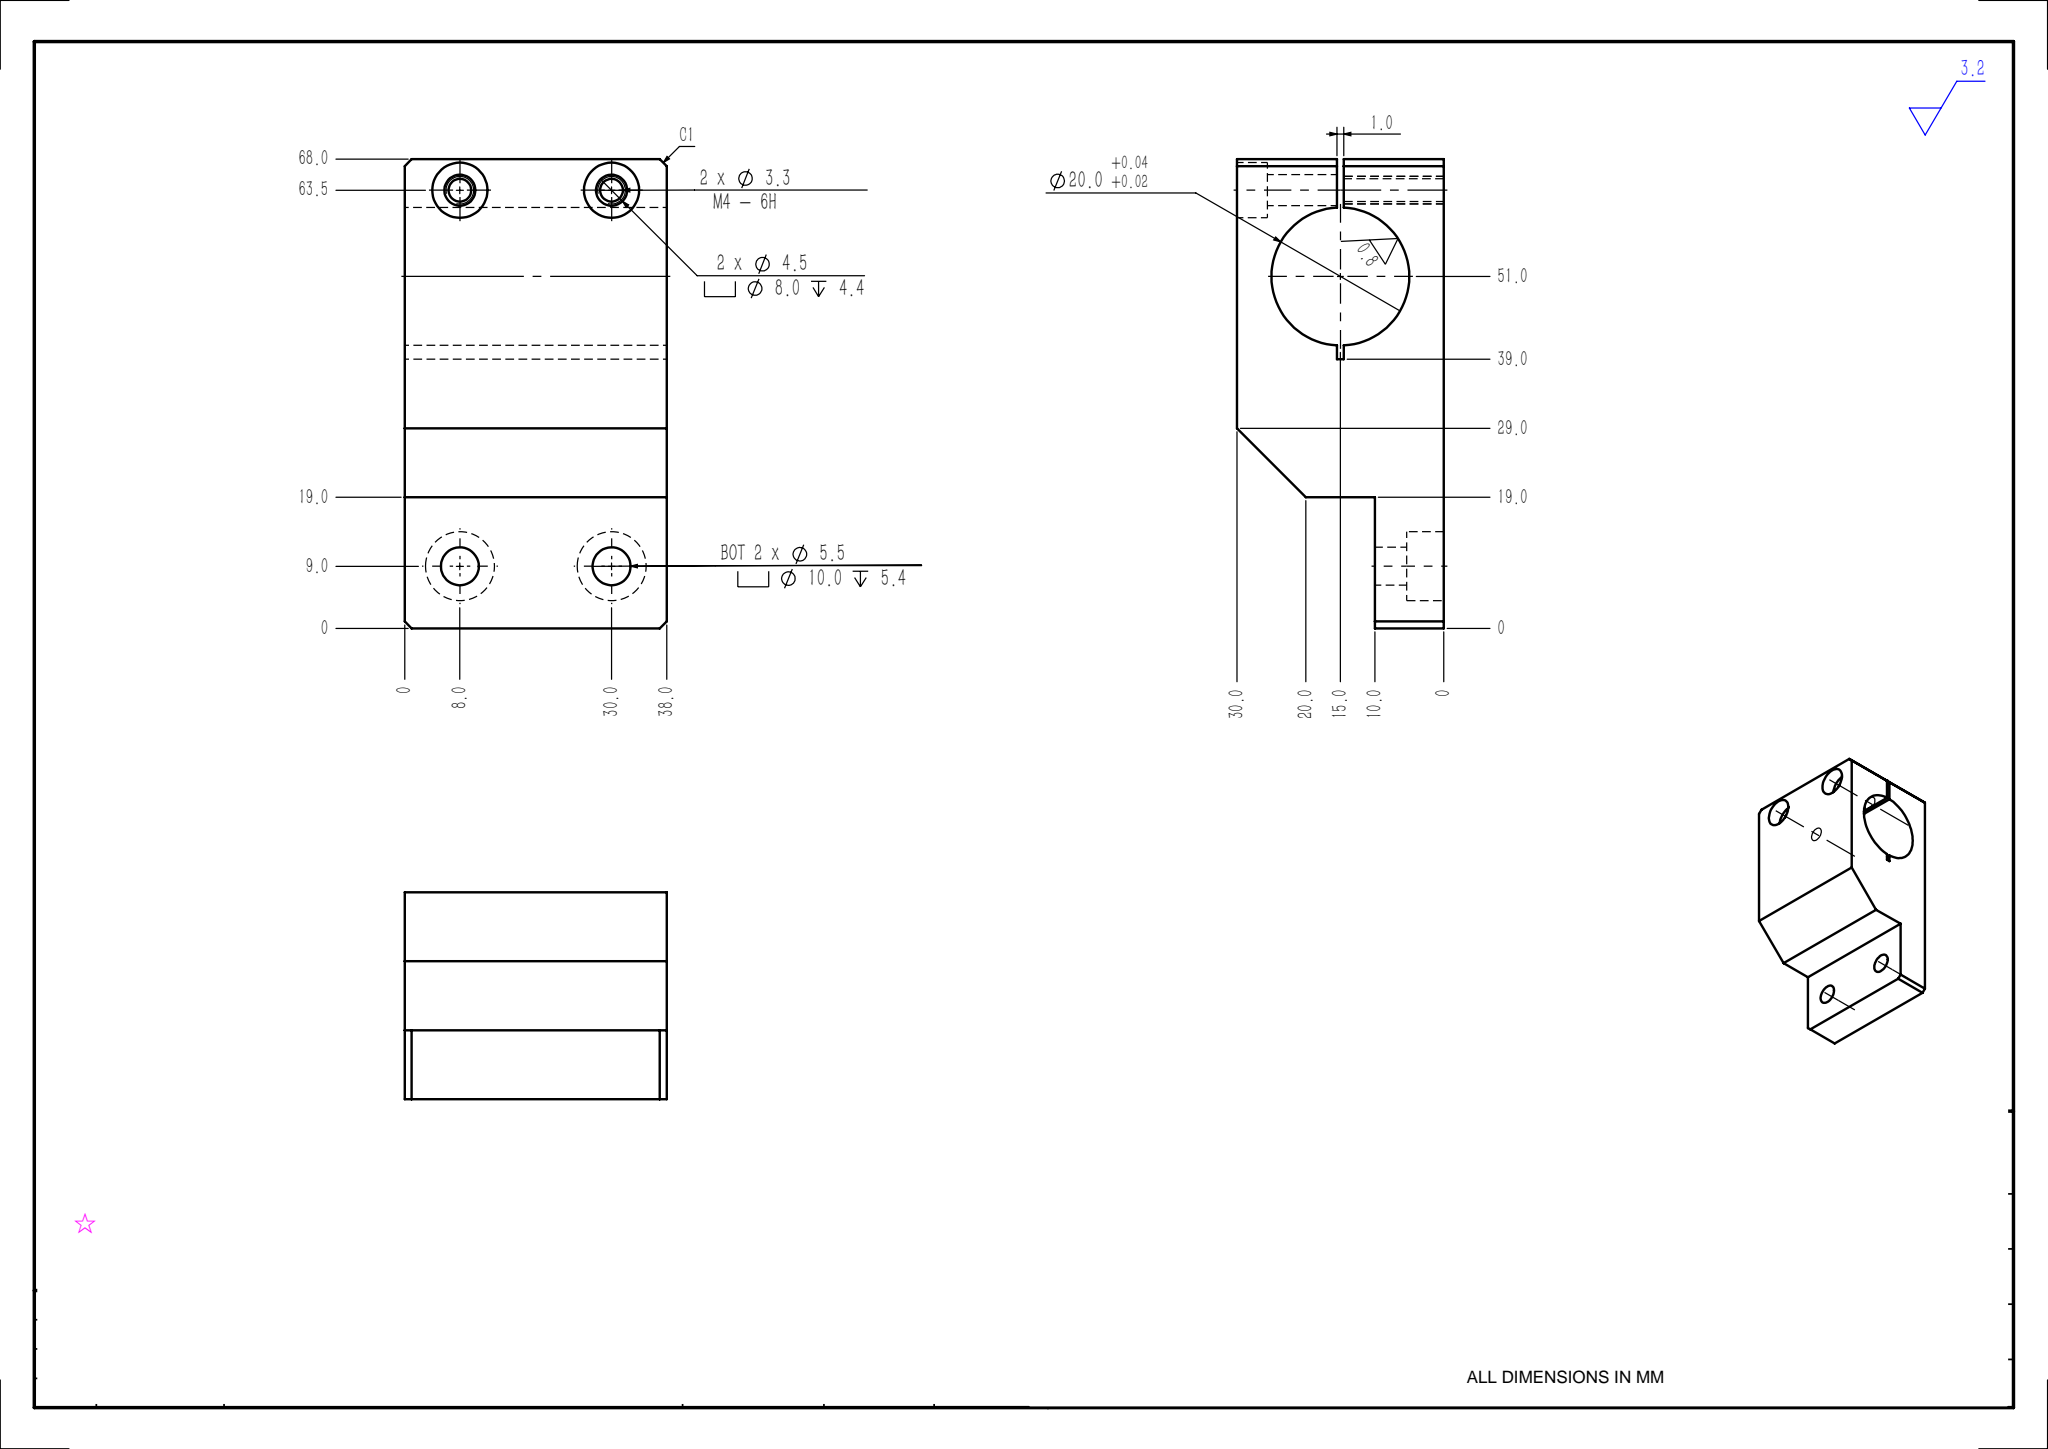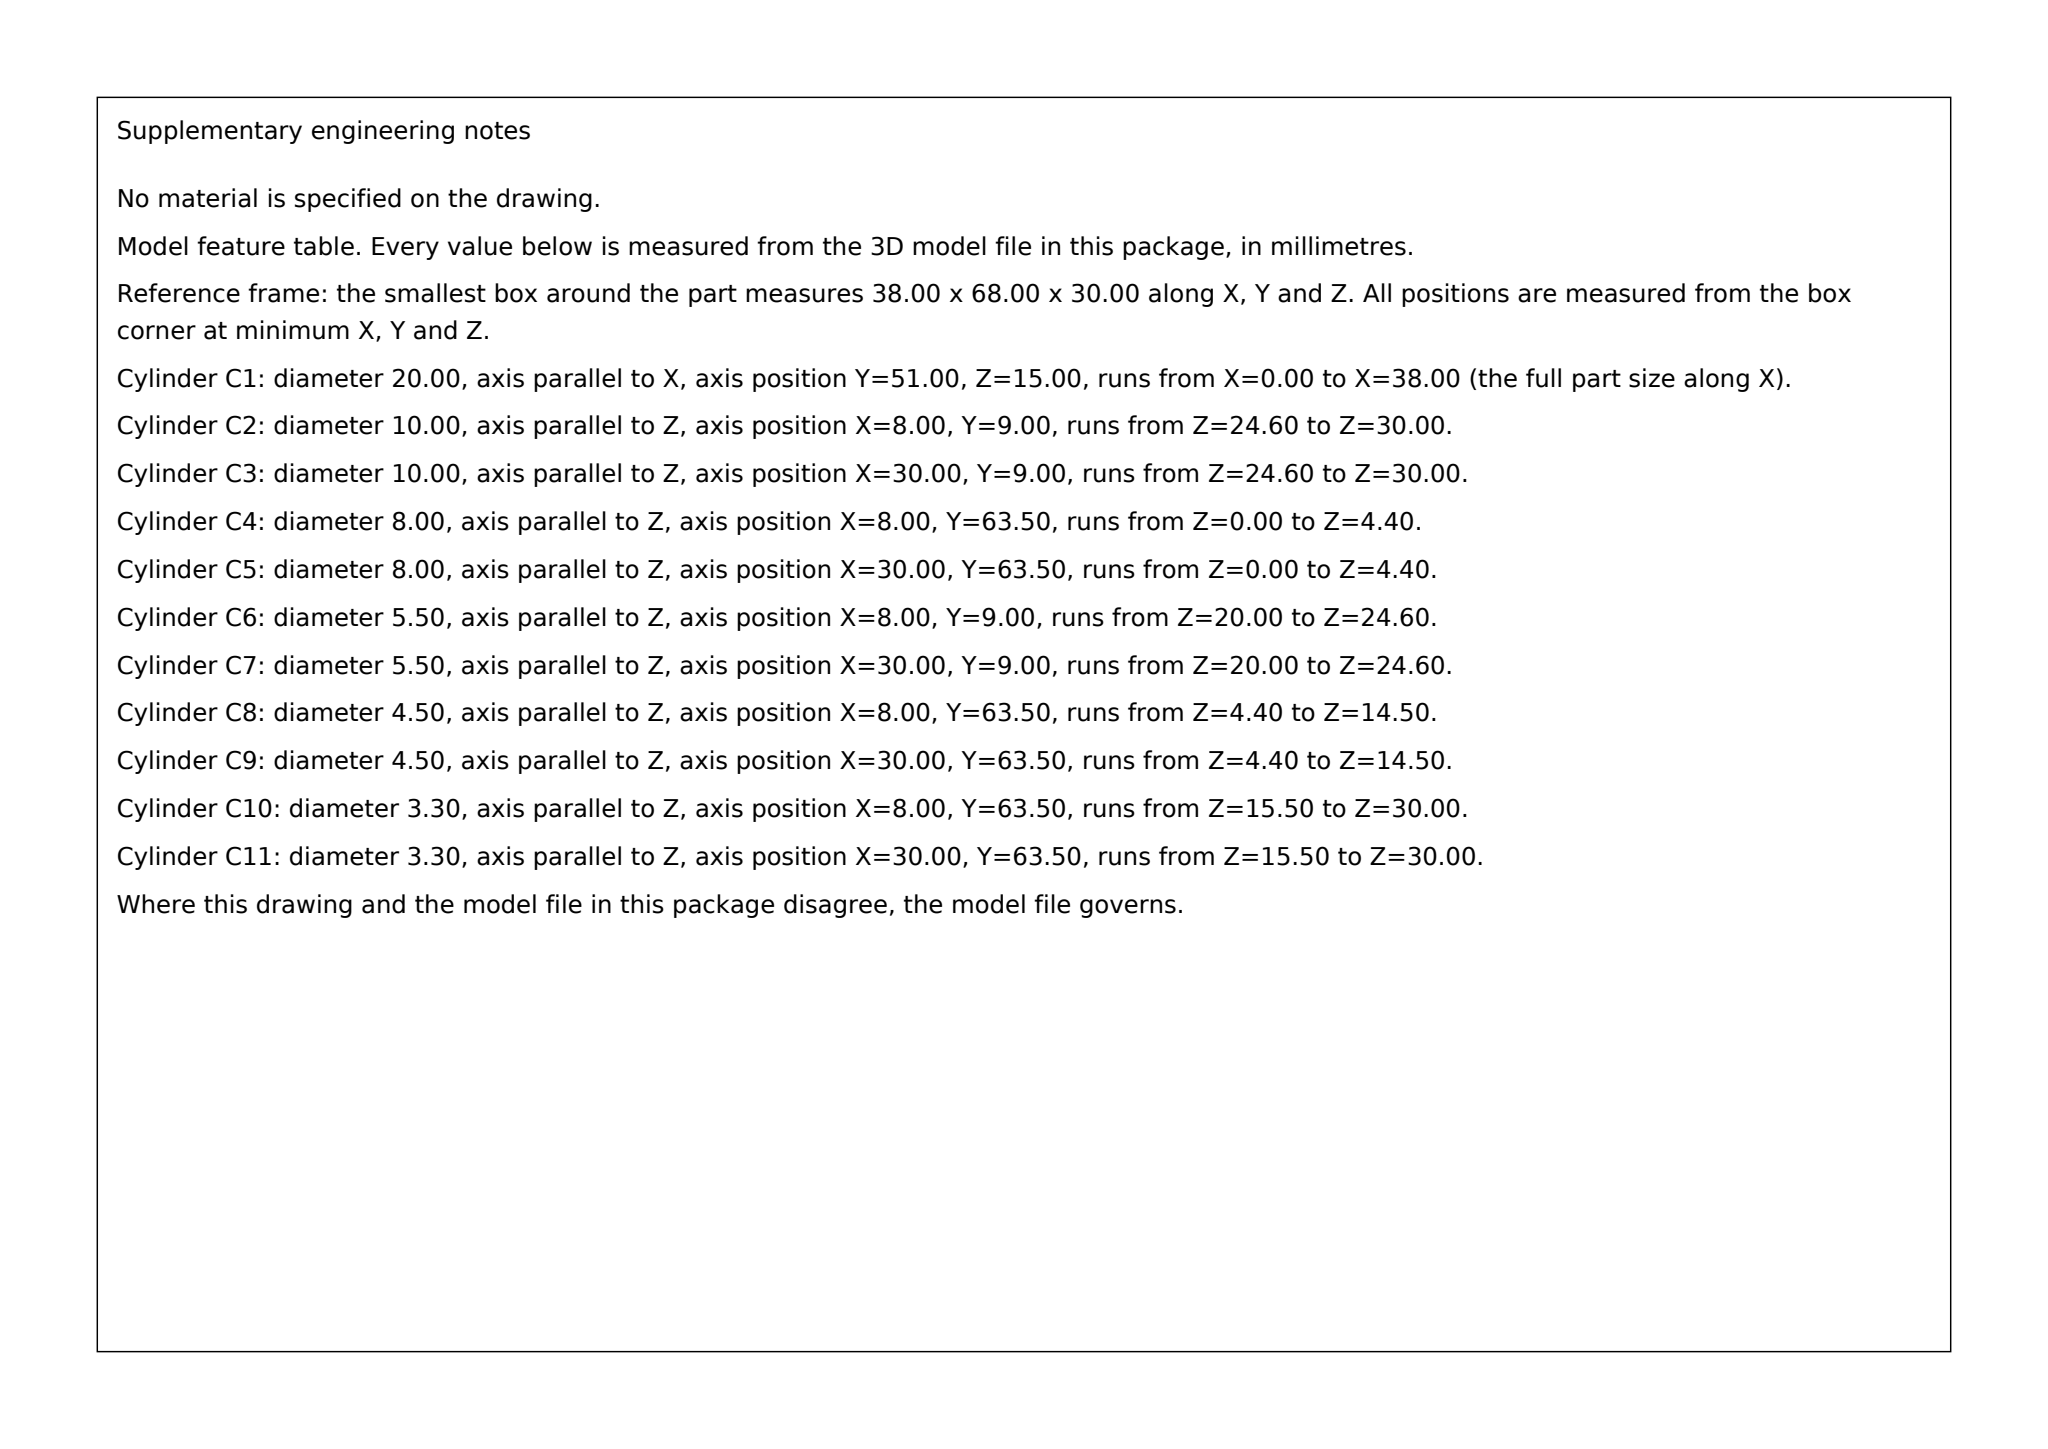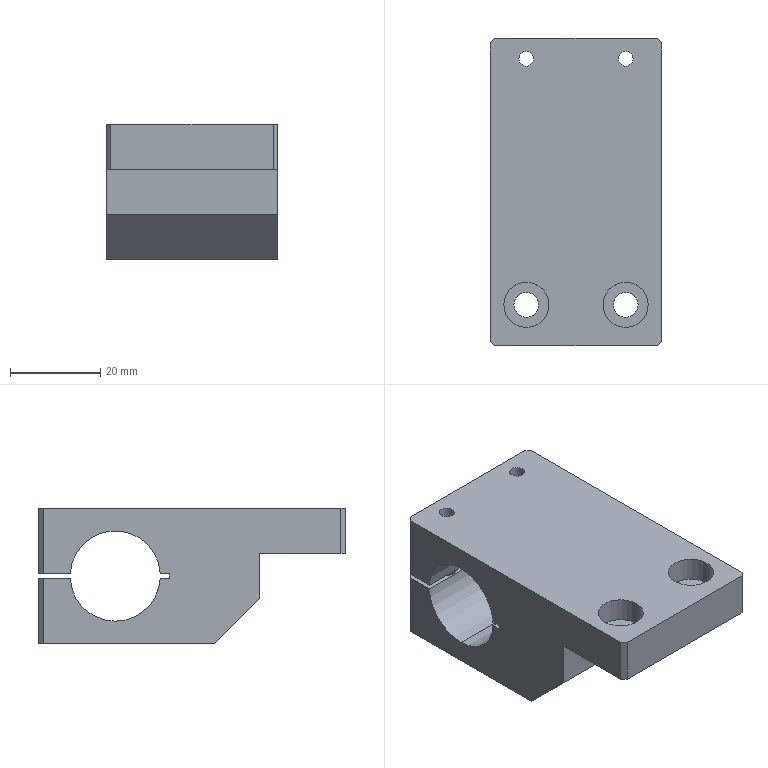Part | SolidWorks | mm | 1 solid | 48 faces | box 38 x 68 x 30 mm | volume 46782 mm3 | plane 25 | cylinder 23 | commonest cylinder face diameters 3.3 x4 8 x4 4.5 x4 10 x4 5.5 x4 20 x3
build123d program:
from build123d import *

# Parameters (mm, degrees)
SKETCH1_W                                       = 38
SKETCH1_H                                       = 68
BOSS_EXTRUDE1_DEPTH                             = 15
SKETCH2_R                                       = 10
CUT_EXTRUDE1_DEPTH                              = 54.151
SKETCH3_W                                       = 1
SKETCH3_H                                       = 29
CUT_EXTRUDE2_DEPTH                              = 54.151
M5_HEX_SOCKET_HEAD_CAP_SCREW_CBORE1_D           = 5.5
M5_HEX_SOCKET_HEAD_CAP_SCREW_CBORE1_CBORE_D     = 10
M5_HEX_SOCKET_HEAD_CAP_SCREW_CBORE1_CBORE_DEPTH = 5.4
M4_HEX_SOCKET_HEAD_CAP_SCREW_CBORE1_D           = 4.5
M4_HEX_SOCKET_HEAD_CAP_SCREW_CBORE1_DEPTH       = 14.5
M4_HEX_SOCKET_HEAD_CAP_SCREW_CBORE1_CBORE_D     = 8
M4_HEX_SOCKET_HEAD_CAP_SCREW_CBORE1_CBORE_DEPTH = 4.4
M4_TAPPED_HOLE1_D                               = 3.3
SKETCH10_W                                      = 38
SKETCH10_H                                      = 19
CUT_EXTRUDE3_DEPTH                              = 20
CHAMFER1_SIZE                                   = 10
CHAMFER2_SIZE                                   = 1


with BuildPart() as part:
    # Sketch1 → Boss-Extrude1 (new, symmetric)
    with BuildSketch(Plane.XY):
        Rectangle(SKETCH1_W, SKETCH1_H)
    extrude(amount=BOSS_EXTRUDE1_DEPTH, both=True)

    # Sketch2 → Cut-Extrude1 (cut, through all)
    with BuildSketch(Plane(origin=(19, 0, 0), x_dir=(0, 0, -1), z_dir=(1, 0, 0))):
        with Locations((0, 17)):
            Circle(SKETCH2_R)
    extrude(amount=-CUT_EXTRUDE1_DEPTH, mode=Mode.SUBTRACT)

    # Sketch3 → Cut-Extrude2 (cut, through all)
    with BuildSketch(Plane(origin=(19, 0, 0), x_dir=(0, 0, -1), z_dir=(1, 0, 0))):
        with Locations((0, 19.5)):
            Rectangle(SKETCH3_W, SKETCH3_H)
    extrude(amount=-CUT_EXTRUDE2_DEPTH, mode=Mode.SUBTRACT)

    # M5 Hex Socket Head Cap Screw CBORE1 (through all)
    with Locations(Plane(origin=(0, 0, 15), x_dir=(-1, 0, 0), z_dir=(0, 0, 1))):
        with Locations((-11, 25), (11, 25)):
            CounterBoreHole(M5_HEX_SOCKET_HEAD_CAP_SCREW_CBORE1_D / 2, M5_HEX_SOCKET_HEAD_CAP_SCREW_CBORE1_CBORE_D / 2, M5_HEX_SOCKET_HEAD_CAP_SCREW_CBORE1_CBORE_DEPTH)

    # M4 Hex Socket Head Cap Screw CBORE1
    with Locations(Plane(origin=(0, 0, -15), x_dir=(-1, 0, 0), z_dir=(0, 0, -1))):
        with Locations((-11, 29.5), (11, 29.5)):
            CounterBoreHole(M4_HEX_SOCKET_HEAD_CAP_SCREW_CBORE1_D / 2, M4_HEX_SOCKET_HEAD_CAP_SCREW_CBORE1_CBORE_D / 2, M4_HEX_SOCKET_HEAD_CAP_SCREW_CBORE1_CBORE_DEPTH, depth=M4_HEX_SOCKET_HEAD_CAP_SCREW_CBORE1_DEPTH)

    # M4 Tapped Hole1 (through all)
    with Locations(Plane(origin=(0, 0, 0.5), x_dir=(-1, 0, 0), z_dir=(0, 0, -1))):
        with Locations((-11, 29.5), (11, 29.5)):
            Hole(M4_TAPPED_HOLE1_D / 2)

    # Sketch10 → Cut-Extrude3 (cut)
    with BuildSketch(Plane(origin=(0, 0, -15), x_dir=(-1, 0, 0), z_dir=(0, 0, -1))):
        with Locations((0, -24.5)):
            Rectangle(SKETCH10_W, SKETCH10_H)
    extrude(amount=-CUT_EXTRUDE3_DEPTH, mode=Mode.SUBTRACT)

    # Chamfer1
    chamfer1_edges = [part.edges().sort_by_distance(p)[0] for p in [
        (0, -15, -15),
    ]]
    chamfer(chamfer1_edges, length=CHAMFER1_SIZE)

    # Chamfer2
    chamfer2_edges = [part.edges().sort_by_distance(p)[0] for p in [
        (-19, 34, -7.75),
        (19, 34, -7.75),
        (19, -34, 10),
        (-19, -34, 10),
        (-19, 34, 7.75),
        (19, 34, 7.75),
    ]]
    chamfer(chamfer2_edges, length=CHAMFER2_SIZE)


solid = part.part